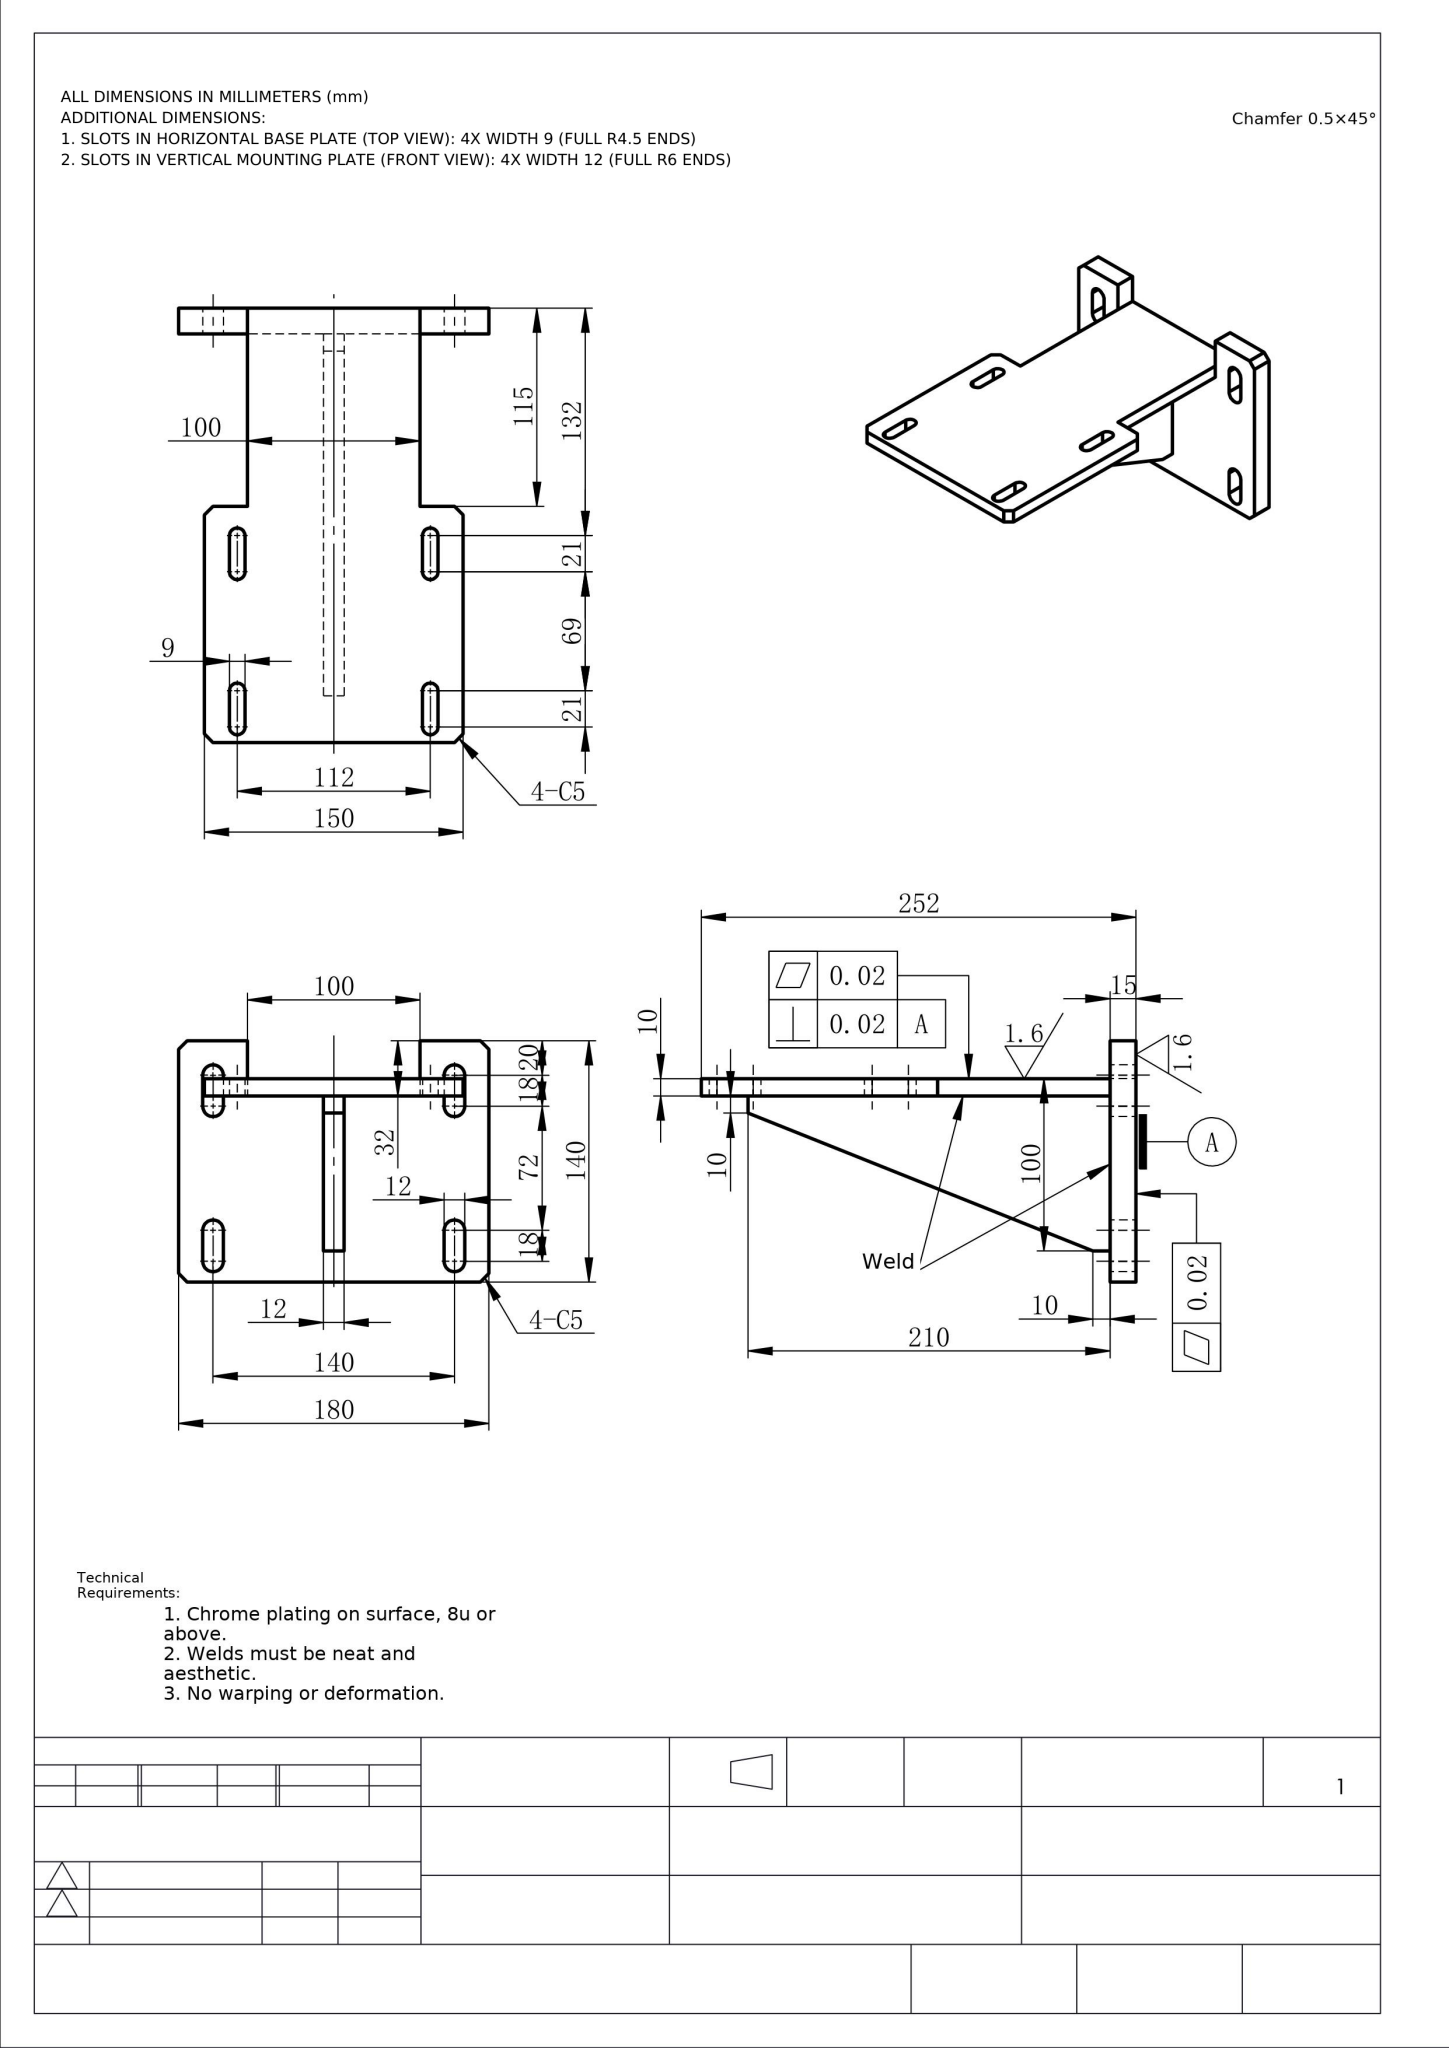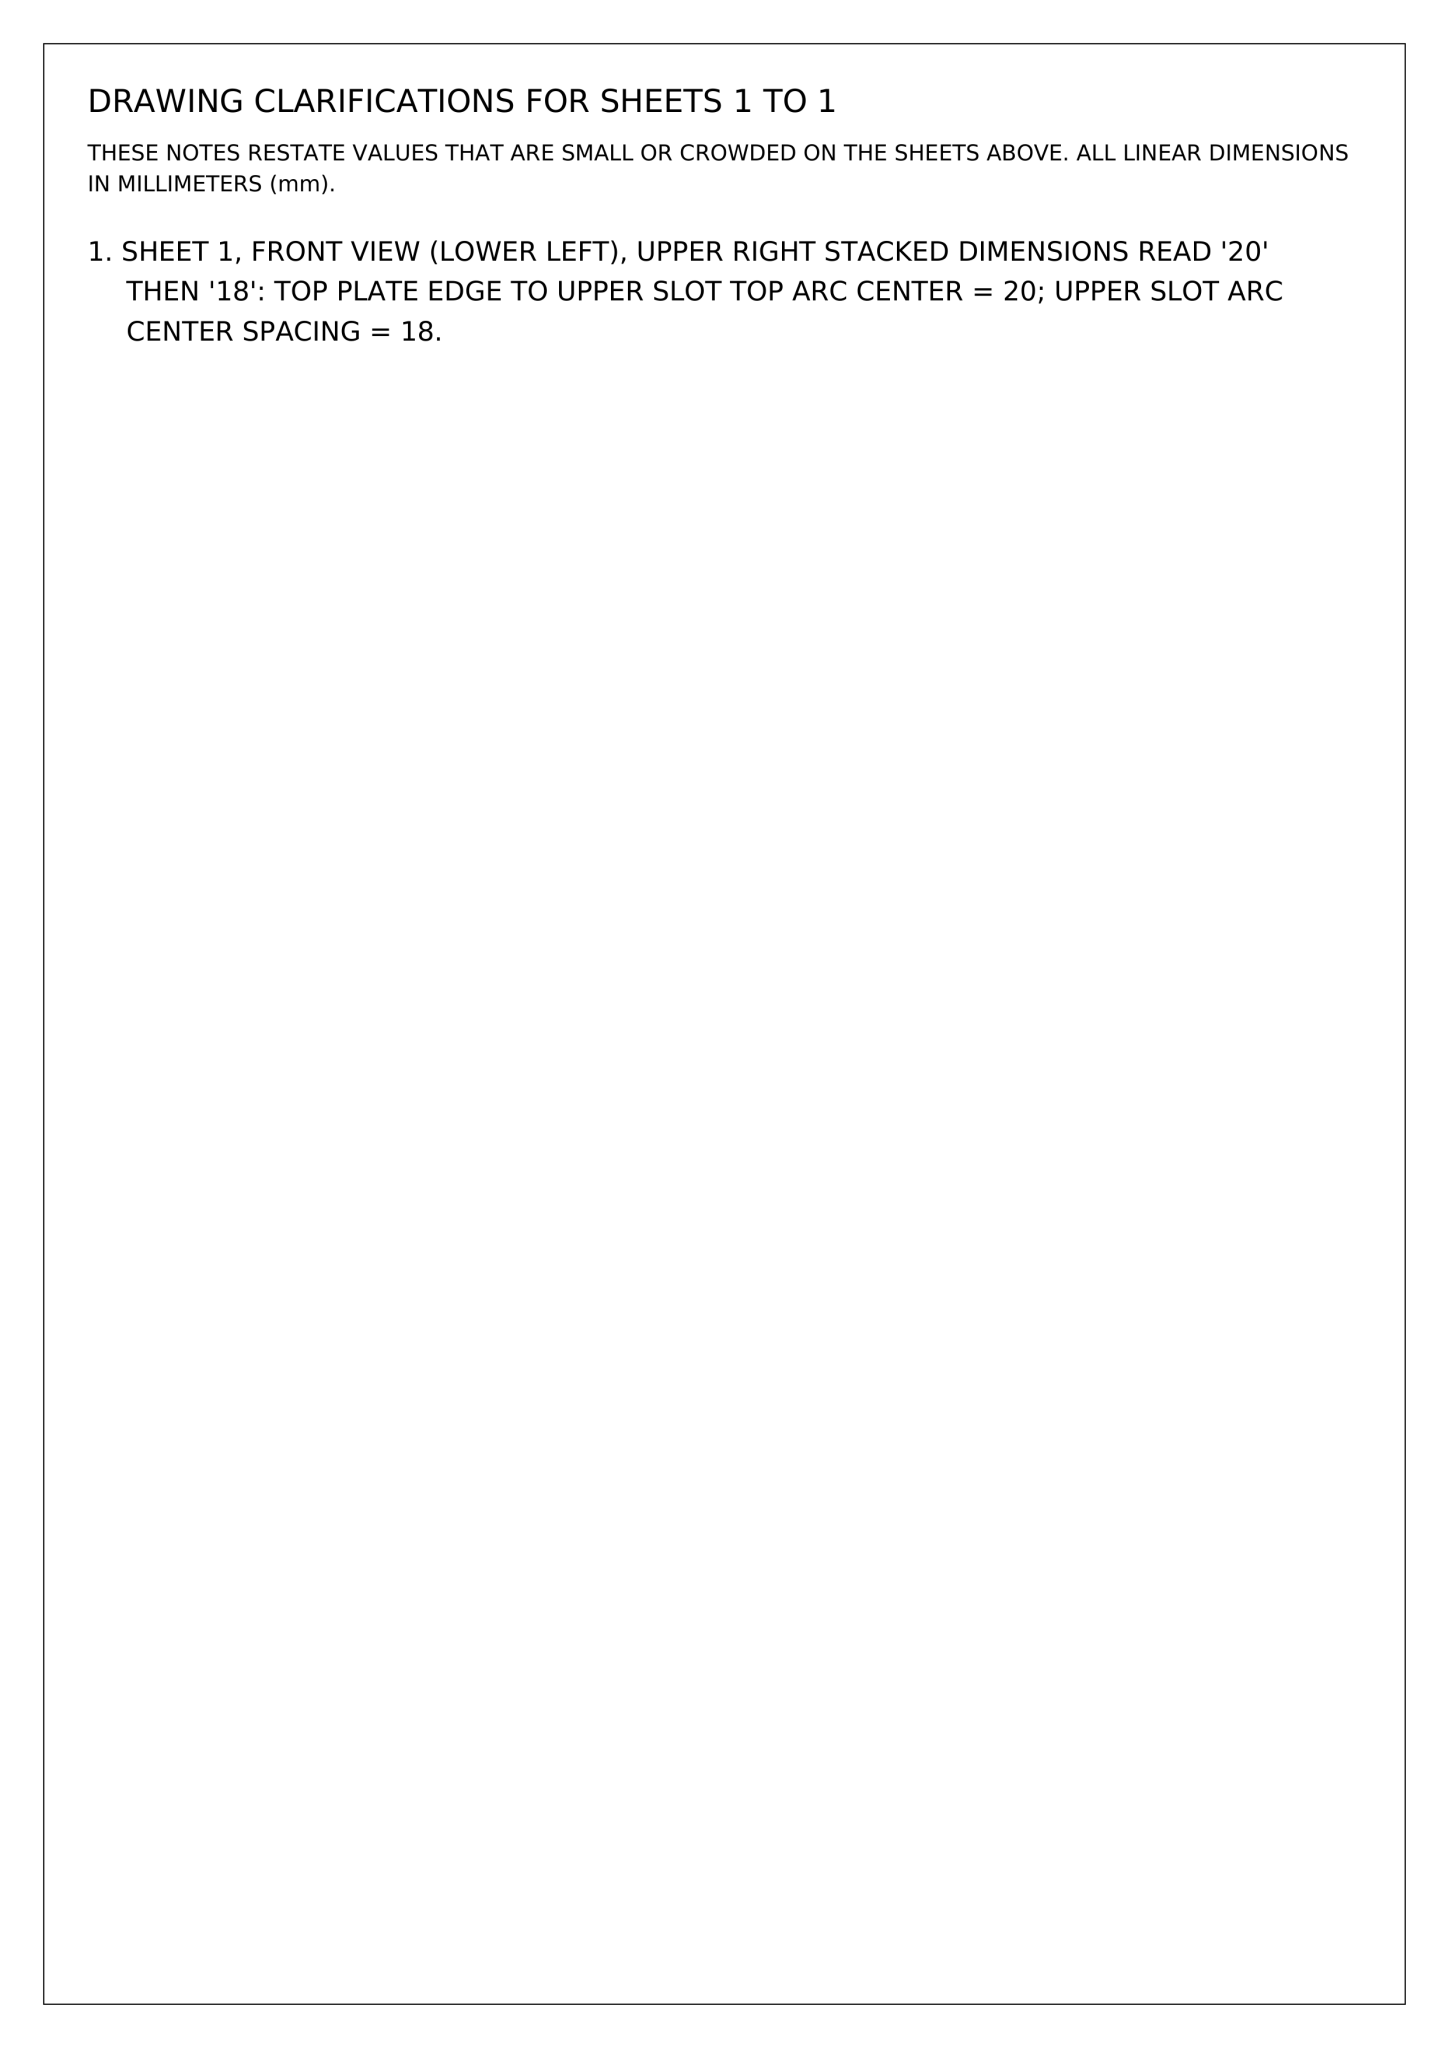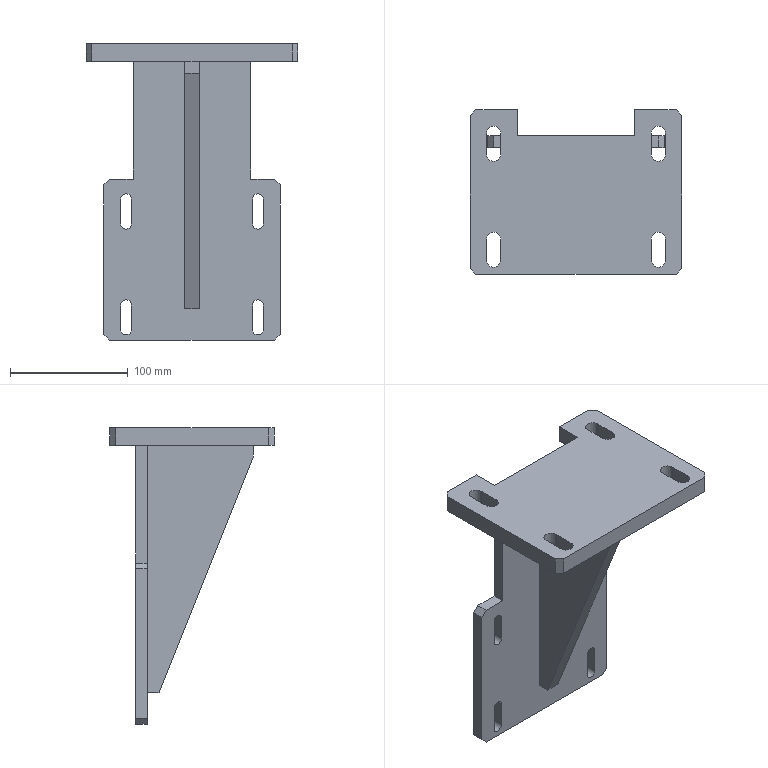Part | NX | mm | 1 solid | 63 faces | box 180 x 140 x 252 mm | volume 750199 mm3 | plane 47 | cylinder 16 | commonest cylinder face diameters 12 x8 9 x8